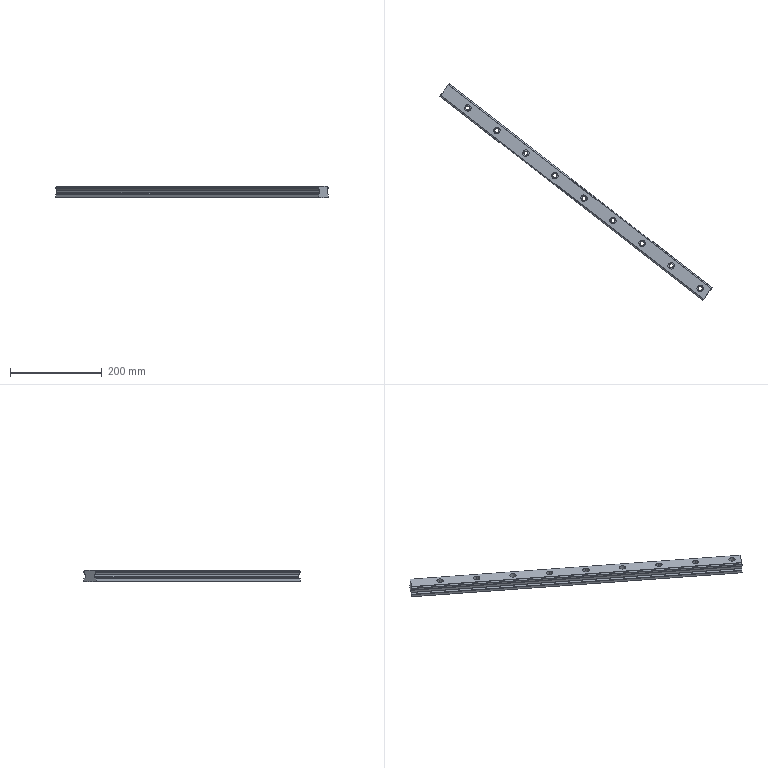Component | SolidWorks | 0803_101_Linear_Guide-1_0803_Z_Linear_Guide_1-1 | 1 solid | 136 faces | box 592.76 x 470.81 x 26 mm | volume 551372 mm3 | cylinder 76 | plane 60 | commonest cylinder face diameters 0.982 x20 14 x18 9 x18 5.719 x4 0.604 x2 0.589 x2 0.6 x2 1.906 x2
build123d program:
from build123d import *

# Parameters (mm, degrees)
BOSS_EXTRUDE1_DEPTH                             = 724
CBORE_FOR_M8_SOCKET_HEAD_CAP_SCREW1_D           = 9
CBORE_FOR_M8_SOCKET_HEAD_CAP_SCREW1_CBORE_D     = 14
CBORE_FOR_M8_SOCKET_HEAD_CAP_SCREW1_CBORE_DEPTH = 12
LPATTERN1_COUNT                                 = 9
LPATTERN1_PITCH                                 = 80


with BuildPart() as part:
    # Sketch1 → Boss-Extrude1 (new body)
    with BuildSketch(Plane(origin=(0, 0, 0), x_dir=(1, 0, 0), z_dir=(0, 1, 0))):
        with BuildLine():
            Line((17, 5.931), (17, 3.069))
            ThreePointArc((17, 3.069), (16.929, 2.874), (16.748, 2.771))
            ThreePointArc((16.748, 2.771), (15.107, 1.931), (14.32, 0.2642))
            ThreePointArc((14.32, 0.2642), (14.223, 0.07565), (14.024, 0))
            Line((14.024, 0), (-14.024, 0))
            ThreePointArc((-14.024, 0), (-14.223, 0.07565), (-14.32, 0.2642))
            ThreePointArc((-14.32, 0.2642), (-15.107, 1.931), (-16.748, 2.771))
            ThreePointArc((-16.748, 2.771), (-16.929, 2.874), (-17, 3.069))
            Line((-17, 3.069), (-17, 5.931))
            ThreePointArc((-17, 5.931), (-16.93, 6.127), (-16.748, 6.227))
            ThreePointArc((-16.748, 6.227), (-15.122, 7.051), (-14.325, 8.69))
            ThreePointArc((-14.325, 8.69), (-14.297, 8.784), (-14.239, 8.864))
            Line((-14.239, 8.864), (-13.796, 9.307))
            ThreePointArc((-13.796, 9.307), (-13.574, 9.63), (-13.5, 10.014))
            Line((-13.5, 10.014), (-13.5, 15.081))
            ThreePointArc((-13.5, 15.081), (-13.577, 15.468), (-13.796, 15.796))
            Line((-13.796, 15.796), (-16.707, 18.707))
            ThreePointArc((-16.707, 18.707), (-16.924, 19.032), (-17, 19.414))
            Line((-17, 19.414), (-17, 24.5))
            Line((-17, 24.5), (-15.5, 26))
            Line((-15.5, 26), (-9.5, 26))
            Line((-9.5, 26), (-9.146, 25.646))
            ThreePointArc((-9.146, 25.646), (-8.984, 25.538), (-8.793, 25.5))
            Line((-8.793, 25.5), (-4.203, 25.5))
            ThreePointArc((-4.203, 25.5), (-4.014, 25.538), (-3.854, 25.646))
            Line((-3.854, 25.646), (-3.5, 26))
            Line((-3.5, 26), (3.5, 26))
            Line((3.5, 26), (3.854, 25.646))
            ThreePointArc((3.854, 25.646), (4.014, 25.538), (4.203, 25.5))
            Line((4.203, 25.5), (8.793, 25.5))
            ThreePointArc((8.793, 25.5), (8.984, 25.538), (9.146, 25.646))
            Line((9.146, 25.646), (9.5, 26))
            Line((9.5, 26), (15.5, 26))
            Line((15.5, 26), (17, 24.5))
            Line((17, 24.5), (17, 19.414))
            ThreePointArc((17, 19.414), (16.924, 19.032), (16.707, 18.707))
            Line((16.707, 18.707), (13.796, 15.796))
            ThreePointArc((13.796, 15.796), (13.577, 15.468), (13.5, 15.081))
            Line((13.5, 15.081), (13.5, 10.014))
            ThreePointArc((13.5, 10.014), (13.574, 9.63), (13.796, 9.307))
            Line((13.796, 9.307), (14.239, 8.864))
            ThreePointArc((14.239, 8.864), (14.297, 8.784), (14.325, 8.69))
            ThreePointArc((14.325, 8.69), (15.122, 7.051), (16.748, 6.227))
            ThreePointArc((16.748, 6.227), (16.93, 6.127), (17, 5.931))
        make_face()
    extrude(amount=BOSS_EXTRUDE1_DEPTH)

    # CBORE for M8 Socket Head Cap Screw1 (through all)
    with Locations(Plane.XY):
        with Locations((0, 20)):
            cbore_for_m8_socket_head_cap_screw1 = CounterBoreHole(CBORE_FOR_M8_SOCKET_HEAD_CAP_SCREW1_D / 2, CBORE_FOR_M8_SOCKET_HEAD_CAP_SCREW1_CBORE_D / 2, CBORE_FOR_M8_SOCKET_HEAD_CAP_SCREW1_CBORE_DEPTH)

    # LPattern1: CBORE for M8 Socket Head Cap Screw1 ×9
    with Locations(*[(0, i * LPATTERN1_PITCH, 0) for i in range(1, LPATTERN1_COUNT)]):
        add(cbore_for_m8_socket_head_cap_screw1, mode=Mode.SUBTRACT)


solid = part.part

# Placed as in the assembly
solid = solid.moved(Location((472.655, 567.626, 327.411), (0, 0, 52.179)))